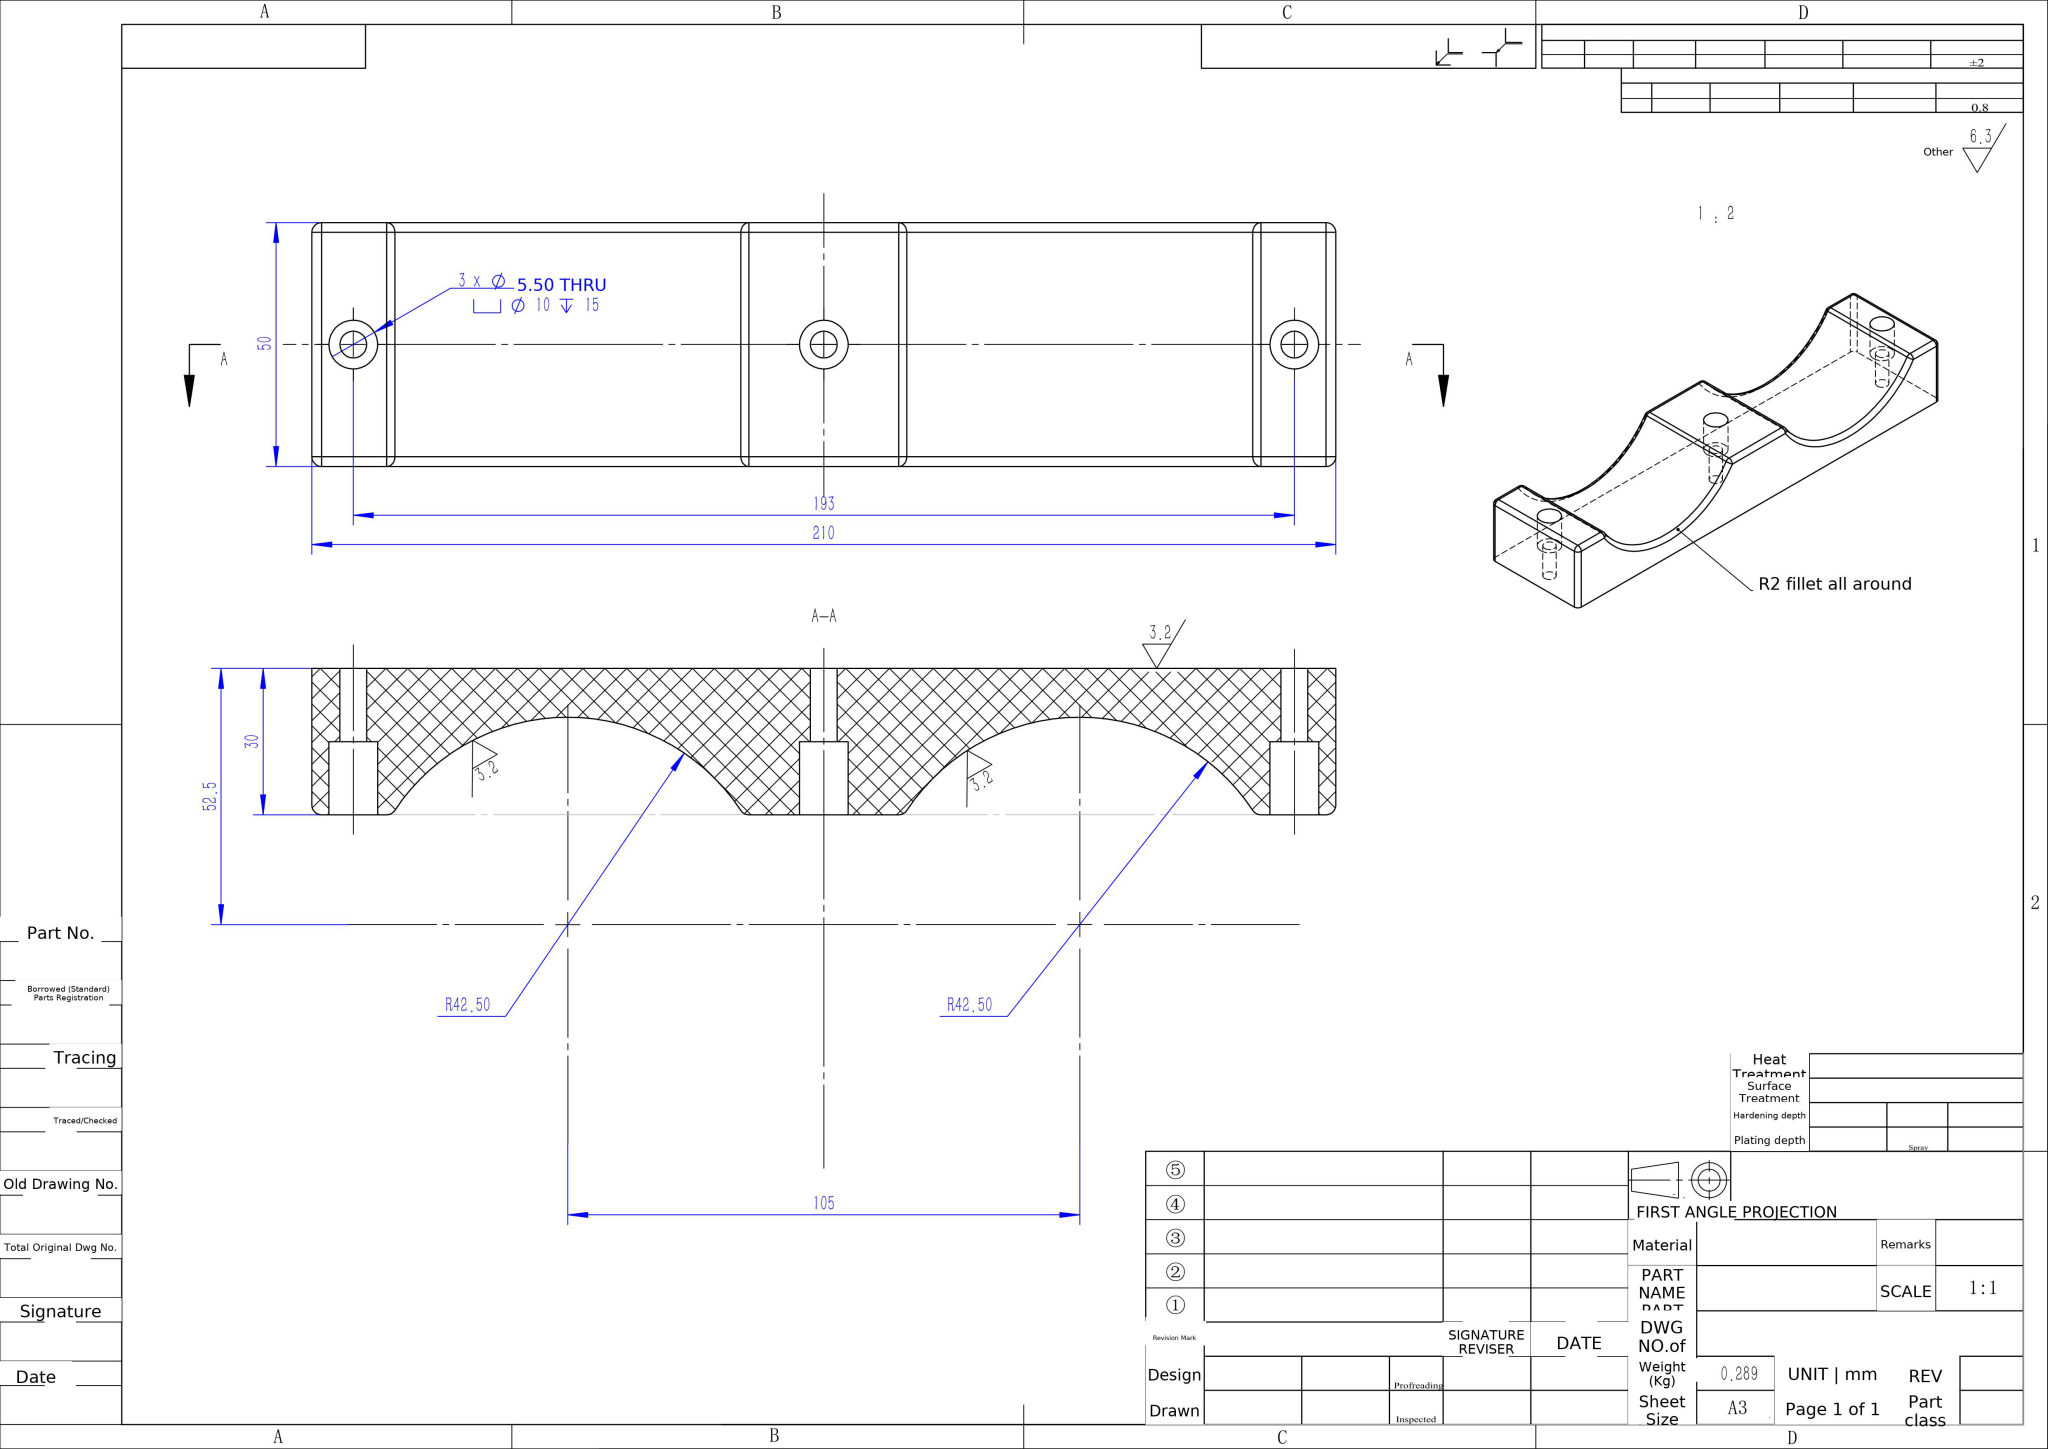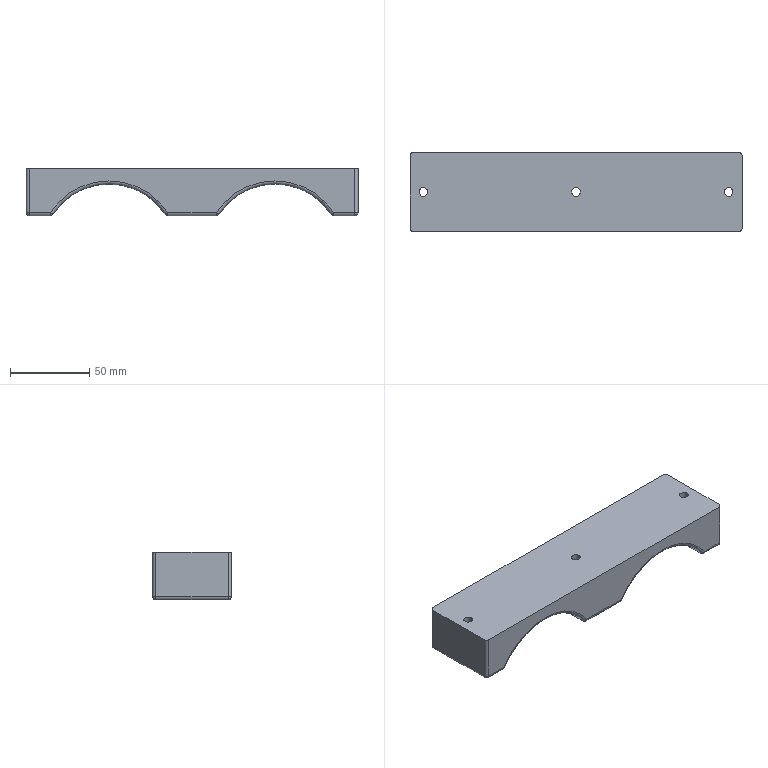Part | NX | mm | 1 solid | 57 faces | box 210 x 50 x 30 mm | volume 207941 mm3 | cylinder 30 | sphere 12 | plane 11 | torus 4 | commonest cylinder face diameters 4 x16 10 x6 5.5 x6 85 x2